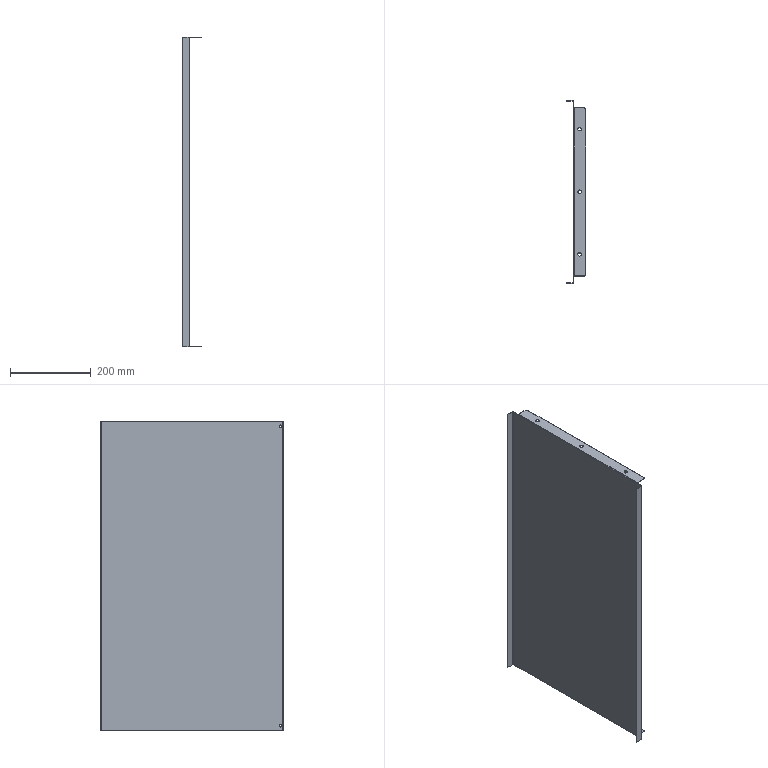Component | SolidWorks | MiddleConnectingPlate-1_MiddleLowerConnectingPlate-1 | 1 solid | 74 faces | volume 319442 mm3 | plane 46 | cylinder 28 | commonest cylinder face diameters 9 x12 6 x4 3.6 x4 2 x4 10 x4 | material 304